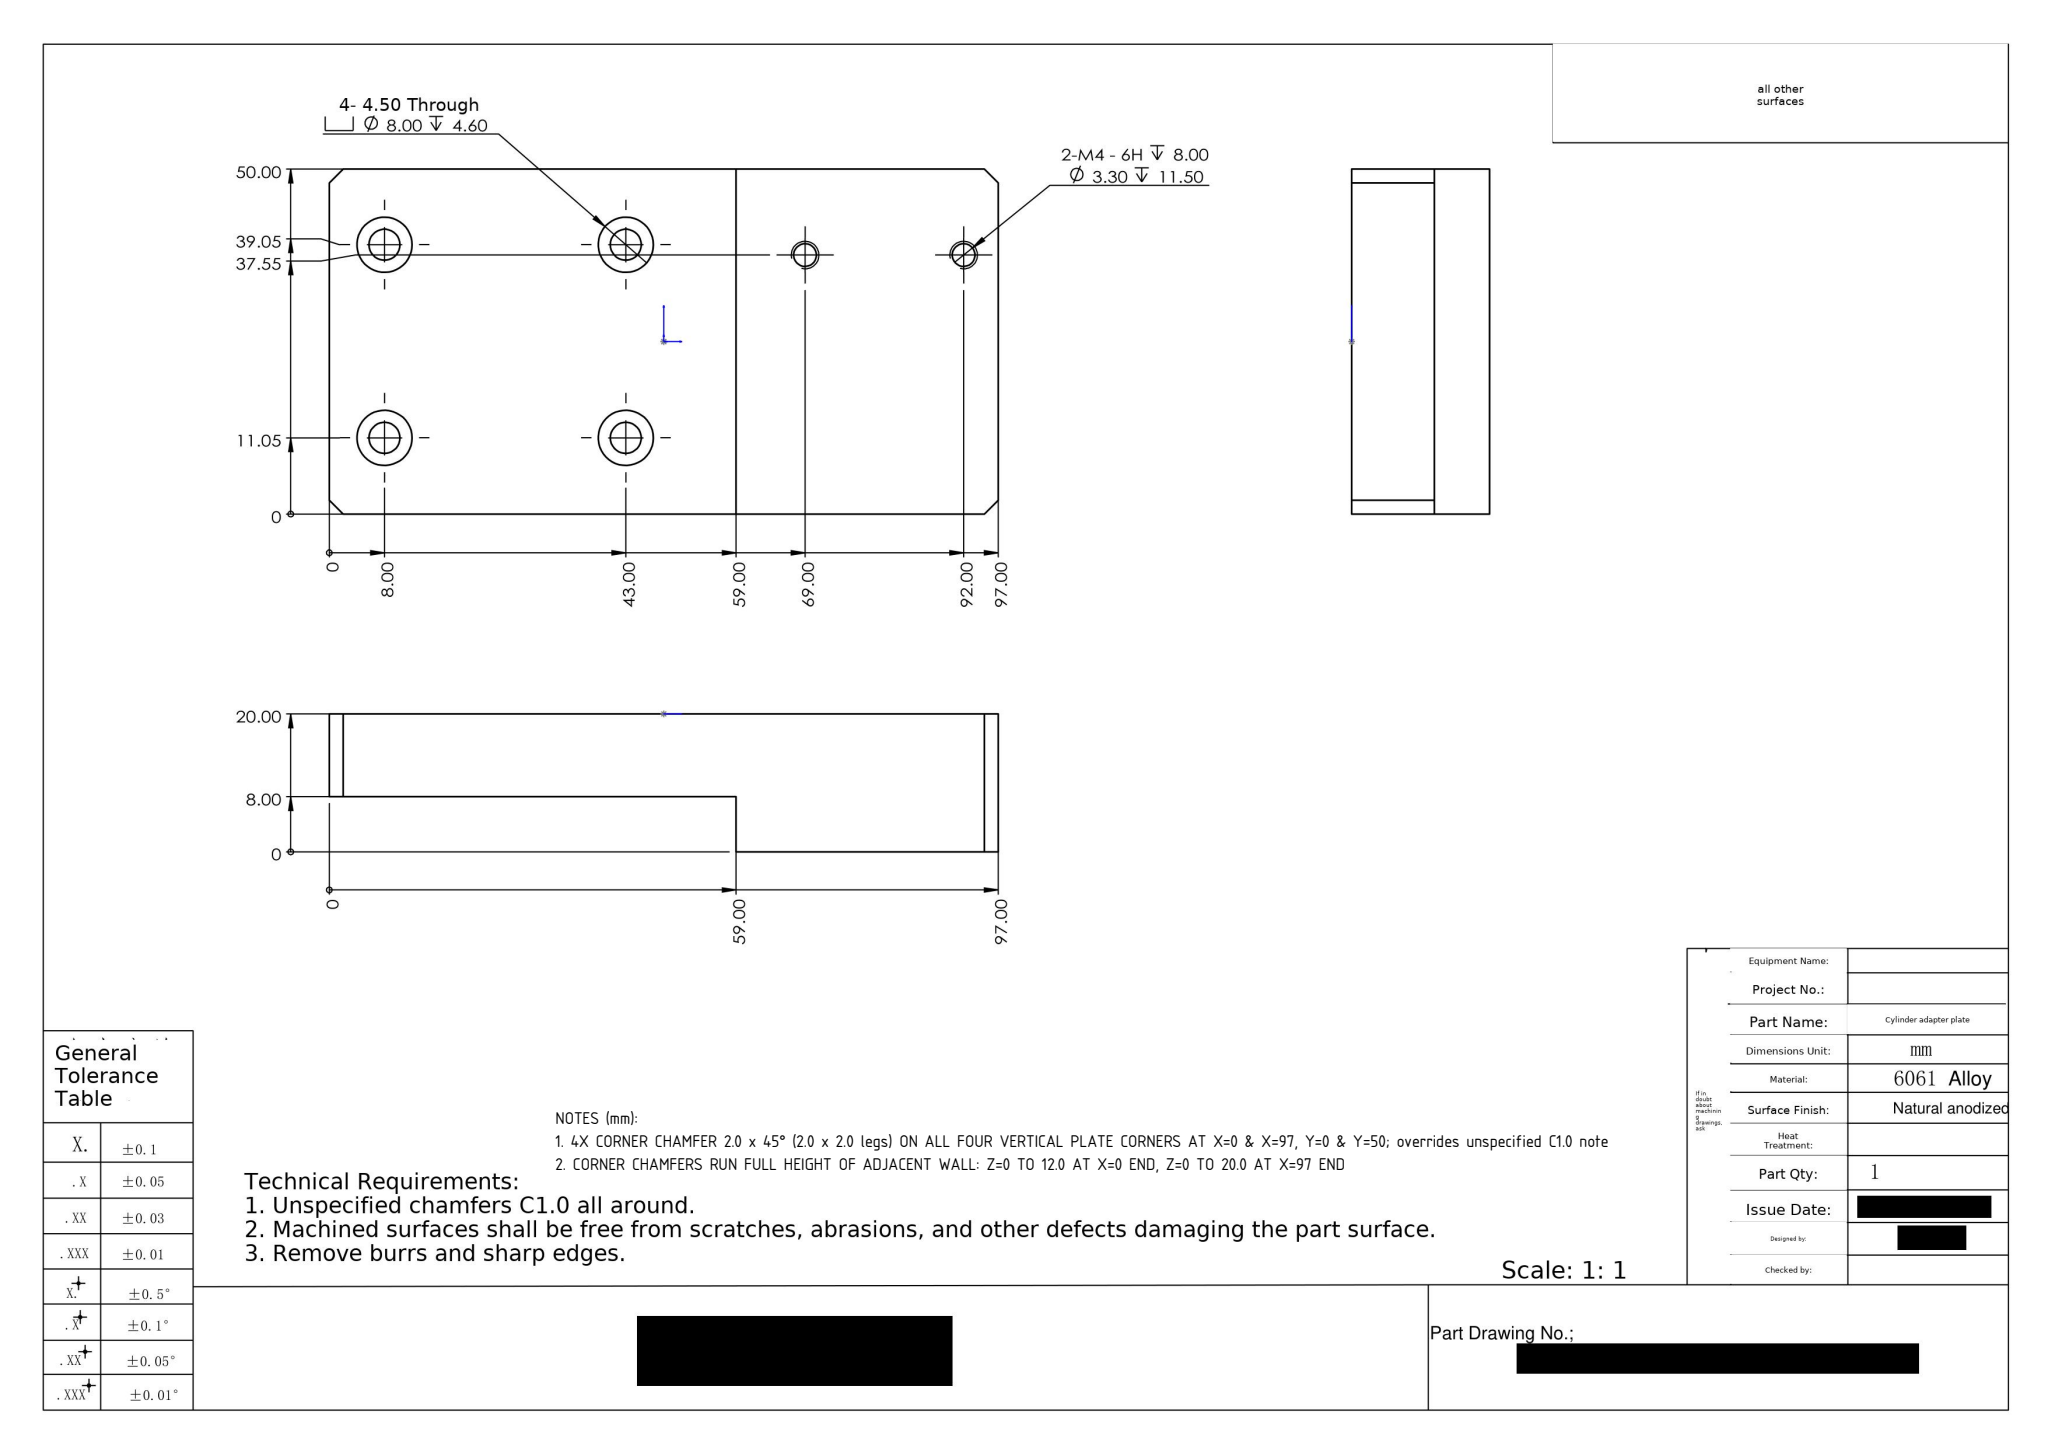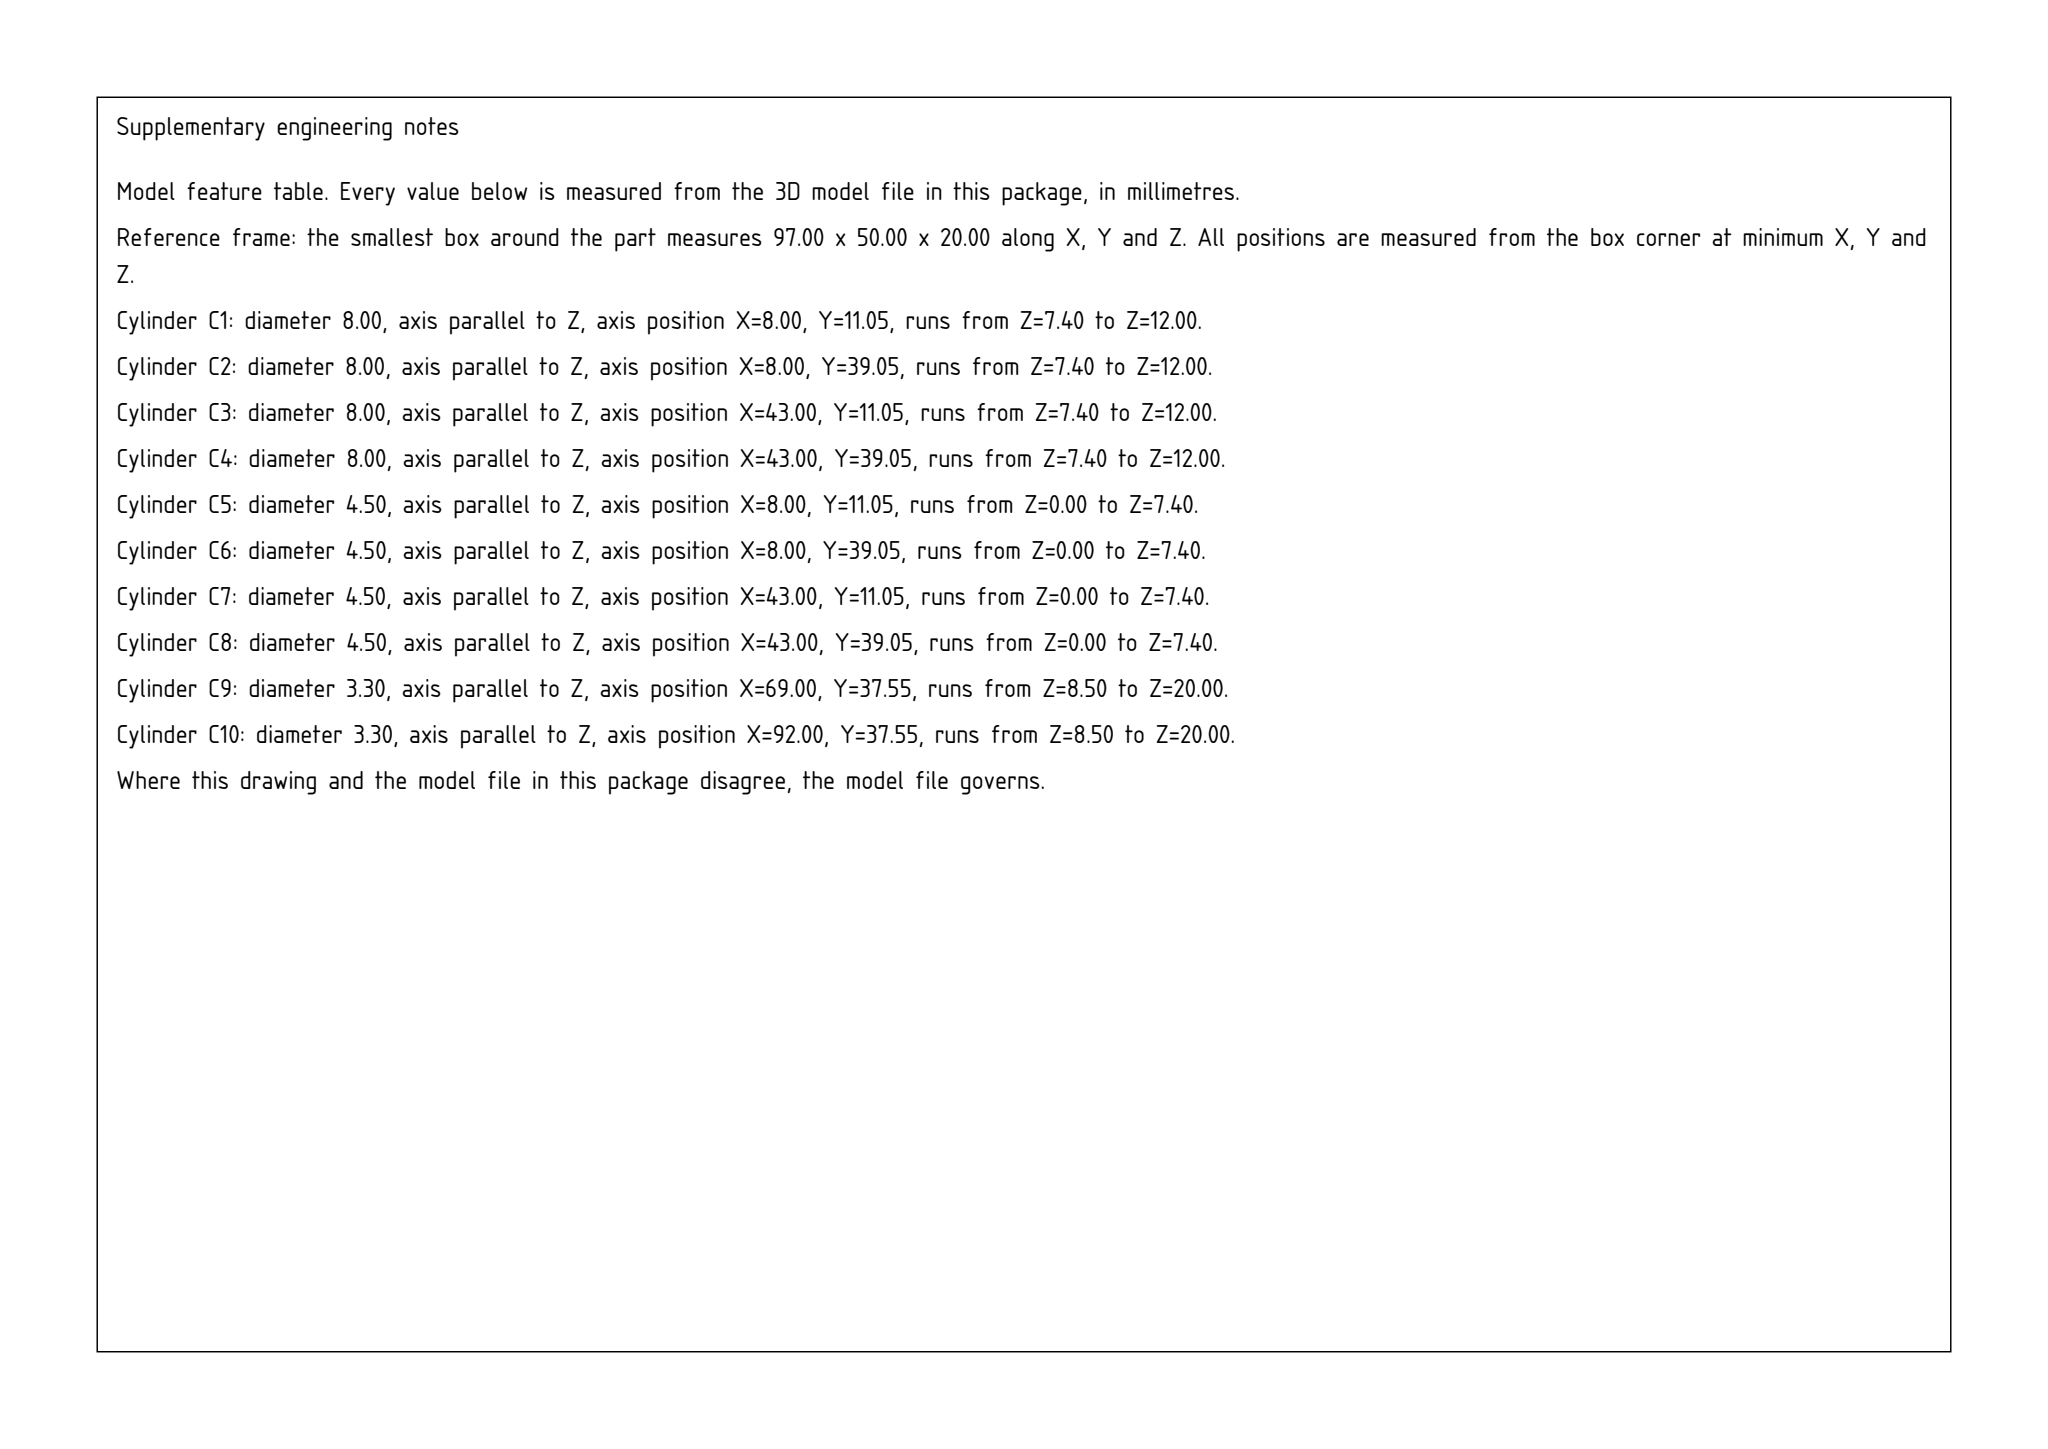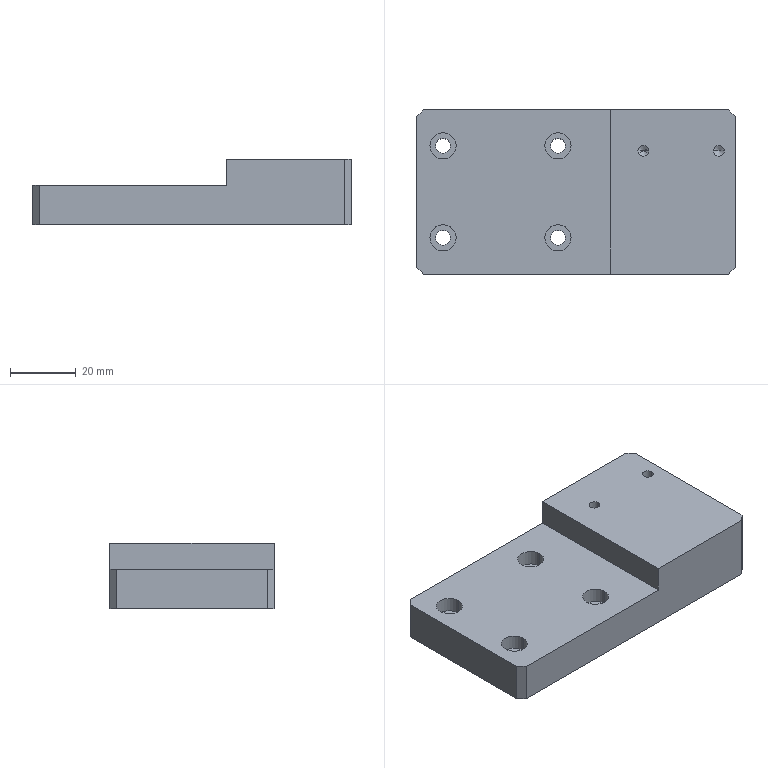Part | SolidWorks | mm | 1 solid | 40 faces | box 97 x 50 x 20 mm | volume 71674 mm3 | cylinder 20 | plane 16 | cone 4 | commonest cylinder face diameters 8 x8 4.5 x8 3.3 x4
Drawing notes:
4X CORNER CHAMFER 2.0 x 45° (2.0 x 2.0 legs) ON ALL FOUR VERTICAL PLATE CORNERS AT X=0 & X=97, Y=0 & Y=50; overrides unspecified C1.0 note | from the solid: inclined_planes: 4 faces at [45.0,45.0,90.0] to XYZ axes, size [2.0,2.0,...] at bbox_from [0,0,0], [0,48,0], [95,0,0], [95,48,0]
CORNER CHAMFERS RUN FULL HEIGHT OF ADJACENT WALL: Z=0 TO 12.0 AT X=0 END, Z=0 TO 20.0 AT X=97 END | from the solid: inclined_planes size Z extent 12.0 at bbox_from X=0 corners and 20.0 at bbox_from X=95 corners; axis_planes x=0 extent z[0,12], x=97 extent z[0,20]
build123d program:
from build123d import *

# Parameters (mm, degrees)
SKETCH1_W                                       = 97
SKETCH1_H                                       = 50
BOSS_EXTRUDE1_DEPTH                             = 20
SKETCH2_W                                       = 59
SKETCH2_H                                       = 50
CUT_EXTRUDE1_DEPTH                              = 8
M4_HEX_SOCKET_HEAD_CAP_SCREW_CBORE1_D           = 4.5
M4_HEX_SOCKET_HEAD_CAP_SCREW_CBORE1_CBORE_D     = 8
M4_HEX_SOCKET_HEAD_CAP_SCREW_CBORE1_CBORE_DEPTH = 4.6
M4_TAPPED_HOLE1_D                               = 3.3
M4_TAPPED_HOLE1_DEPTH                           = 11.5
M4_TAPPED_HOLE1_TIP                             = 0.9914
CHAMFER1_SIZE                                   = 2


with BuildPart() as part:
    # Sketch1 → Boss-Extrude1 (new body)
    with BuildSketch(Plane.XY):
        Rectangle(SKETCH1_W, SKETCH1_H)
    extrude(amount=BOSS_EXTRUDE1_DEPTH)

    # Sketch2 → Cut-Extrude1 (cut)
    with BuildSketch(Plane.XY.offset(20)):
        with Locations((-19, 0)):
            Rectangle(SKETCH2_W, SKETCH2_H)
    extrude(amount=-CUT_EXTRUDE1_DEPTH, mode=Mode.SUBTRACT)

    # M4 Hex Socket Head Cap Screw CBORE1 (through all)
    with Locations(Plane.XY.offset(12)):
        with Locations((-5.5, -13.95), (-40.5, -13.95), (-5.5, 14.05), (-40.5, 14.05)):
            CounterBoreHole(M4_HEX_SOCKET_HEAD_CAP_SCREW_CBORE1_D / 2, M4_HEX_SOCKET_HEAD_CAP_SCREW_CBORE1_CBORE_D / 2, M4_HEX_SOCKET_HEAD_CAP_SCREW_CBORE1_CBORE_DEPTH)

    # M4 Tapped Hole1
    with Locations(Plane.XY.offset(20)):
        with Locations((43.5, 12.55), (20.5, 12.55)):
            Hole(M4_TAPPED_HOLE1_D / 2, depth=M4_TAPPED_HOLE1_DEPTH)
            with Locations((0, 0, -(M4_TAPPED_HOLE1_DEPTH + M4_TAPPED_HOLE1_TIP / 2))):  # 118° drill point
                Cone(0, M4_TAPPED_HOLE1_D / 2, M4_TAPPED_HOLE1_TIP, mode=Mode.SUBTRACT)

    # Chamfer1
    chamfer1_edges = [part.edges().sort_by_distance(p)[0] for p in [
        (-48.5, -25, 6),
        (-48.5, 25, 6),
        (48.5, -25, 10),
        (48.5, 25, 10),
    ]]
    chamfer(chamfer1_edges, length=CHAMFER1_SIZE)


solid = part.part